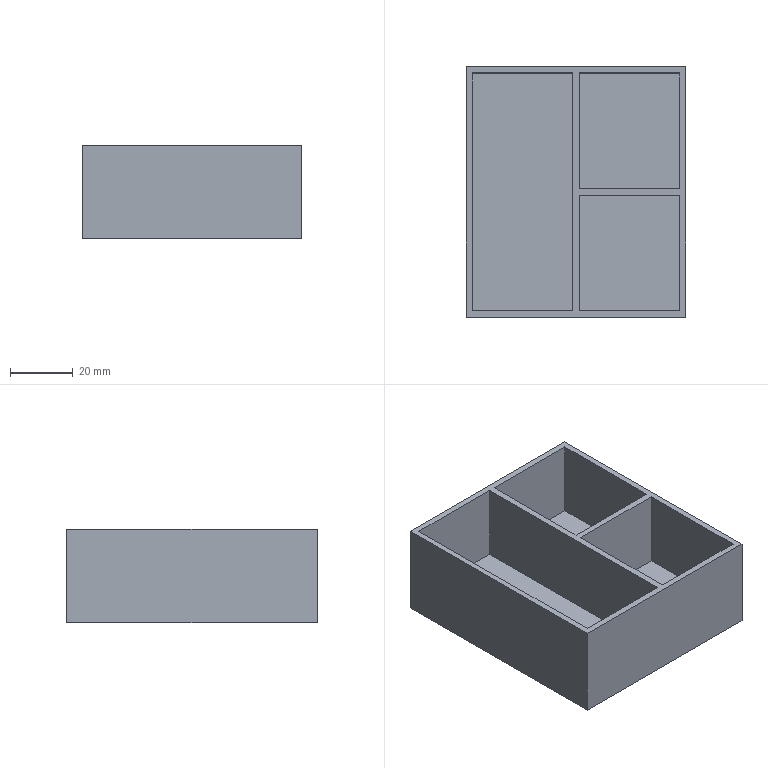Component | NX | REMOVABLE_STORAGE_2 | 1 solid | 21 faces | volume 48000 mm3 | plane 21